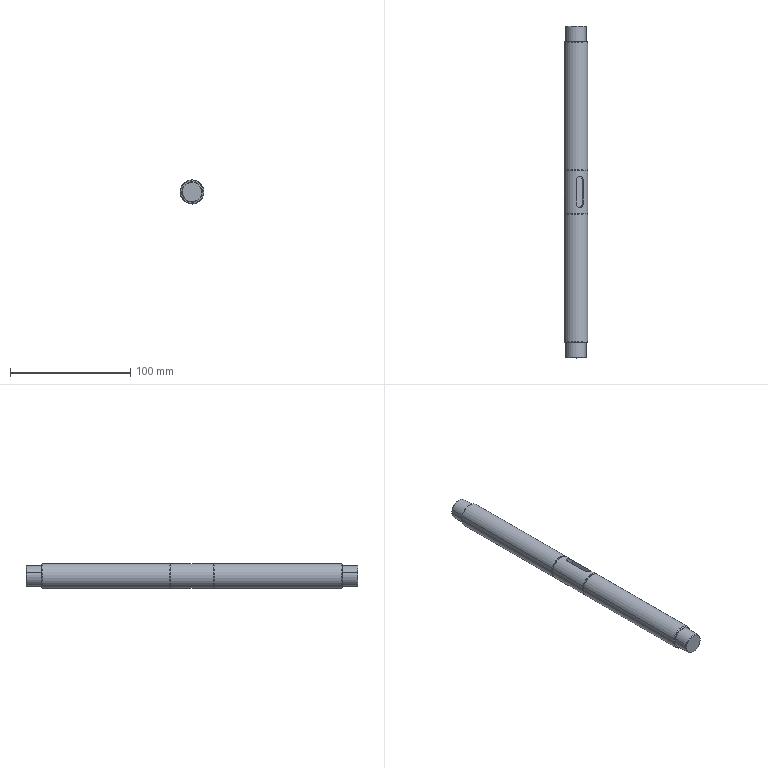Component | SolidWorks | CTM-T-12-D-GD-03-1 | 1 solid | 36 faces | box 20 x 276 x 20 mm | volume 83848 mm3 | cylinder 17 | plane 11 | cone 8 | commonest cylinder face diameters 20 x6 17 x4 19 x4 6 x3 | material 45
build123d program:
from build123d import *

# Parameters (mm, degrees)
SKETCH1_R           = 10
BOSS_EXTRUDE1_DEPTH = 125
SKETCH2_R           = 8.5
BOSS_EXTRUDE2_DEPTH = 13
BOSS_EXTRUDE3_START = 13
SKETCH3_R           = 8.5
BOSS_EXTRUDE3_DEPTH = 13
CUT_EXTRUDE2_DEPTH  = 3.5
CHAMFER1_SIZE       = 0.5
CHAMFER2_SIZE       = 0.5
SKETCH8_R           = 10
SKETCH8_R_2         = 9.5
CUT_EXTRUDE3_DEPTH  = 1.1


with BuildPart() as part:
    # Sketch1 → Boss-Extrude1 (new, symmetric)
    with BuildSketch(Plane.XY):
        Circle(SKETCH1_R)
    extrude(amount=BOSS_EXTRUDE1_DEPTH, both=True)

    # Sketch2 → Boss-Extrude2 (add)
    with BuildSketch(Plane(origin=(0, 0, -125), x_dir=(-1, 0, 0), z_dir=(0, 0, -1))):
        with Locations(Location((0, 0, 0), (0, 0, 180))):
            Circle(SKETCH2_R)
    extrude(amount=BOSS_EXTRUDE2_DEPTH)

    # Sketch3 → Boss-Extrude3 (add)
    with BuildSketch(Plane.XY.offset(125).offset(BOSS_EXTRUDE3_START)):
        Circle(SKETCH3_R)
    extrude(amount=-BOSS_EXTRUDE3_DEPTH)

    # Sketch7 → Cut-Extrude2 (cut)
    with BuildSketch(Plane(origin=(0, 10, 0), x_dir=(-1, 0, 0), z_dir=(0, 1, 0))):
        with BuildLine():
            Line((3, 10), (3, -10))
            ThreePointArc((3, -10), (0, -13), (-3, -10))
            Line((-3, -10), (-3, 10))
            ThreePointArc((-3, 10), (0, 13), (3, 10))
        make_face()
    extrude(amount=-CUT_EXTRUDE2_DEPTH, mode=Mode.SUBTRACT)

    # Chamfer1
    chamfer1_edges = [part.edges().sort_by_distance(p)[0] for p in [
        (-8.5, 0, 138),
        (-8.5, 0, -138),
    ]]
    chamfer(chamfer1_edges, length=CHAMFER1_SIZE)

    # Chamfer2
    chamfer2_edges = [part.edges().sort_by_distance(p)[0] for p in [
        (-10, 0, -125),
        (-10, 0, 125),
    ]]
    chamfer(chamfer2_edges, length=CHAMFER2_SIZE)

    # Sketch8 → Cut-Extrude3 (cut)
    with BuildSketch(Plane.XY.offset(18.65)):
        Circle(SKETCH8_R)
        Circle(SKETCH8_R_2, mode=Mode.SUBTRACT)
    cut_extrude3 = extrude(amount=-CUT_EXTRUDE3_DEPTH, mode=Mode.SUBTRACT)

    # Mirror1: Cut-Extrude3 across plane
    add(cut_extrude3.mirror(Plane.XY), mode=Mode.SUBTRACT)


solid = part.part

# Placed as in the assembly
solid = solid.moved(Location((40.4, -145, 35), (-90, 0, -160.666)))
STEP:
#1=CARTESIAN_POINT('',(1.962,-4.974,1.248));
#2=VERTEX_POINT('',#1);
#3=CARTESIAN_POINT('',(1.219,-4.974,1.508));
#4=VERTEX_POINT('',#3);
#5=CARTESIAN_POINT('',(1.591,-4.974,1.378));
#6=DIRECTION('',(-0.,-1.,-0.));
#7=DIRECTION('',(0.9436,0.,-0.3311));
#8=AXIS2_PLACEMENT_3D('',#5,#6,#7);
#9=CIRCLE('',#8,0.3937);
#10=EDGE_CURVE('',#2,#4,#9,.T.);
#11=ORIENTED_EDGE('',*,*,#10,.F.);
#12=CARTESIAN_POINT('',(1.962,-0.8071,1.248));
#13=VERTEX_POINT('',#12);
#14=CARTESIAN_POINT('',(1.962,-10.63,1.248));
#15=DIRECTION('',(0.,1.,0.));
#16=VECTOR('',#15,39.37);
#17=LINE('',#14,#16);
#18=EDGE_CURVE('',#2,#13,#17,.T.);
#19=ORIENTED_EDGE('',*,*,#18,.T.);
#20=CARTESIAN_POINT('',(1.219,-0.8071,1.508));
#21=VERTEX_POINT('',#20);
#22=CARTESIAN_POINT('',(1.591,-0.8071,1.378));
#23=DIRECTION('',(-0.,-1.,-0.));
#24=DIRECTION('',(0.9436,0.,-0.3311));
#25=AXIS2_PLACEMENT_3D('',#22,#23,#24);
#26=CIRCLE('',#25,0.3937);
#27=EDGE_CURVE('',#13,#21,#26,.T.);
#28=ORIENTED_EDGE('',*,*,#27,.T.);
#29=CARTESIAN_POINT('',(1.219,-10.63,1.508));
#30=DIRECTION('',(0.,1.,0.));
#31=VECTOR('',#30,39.37);
#32=LINE('',#29,#31);
#33=EDGE_CURVE('',#4,#21,#32,.T.);
#34=ORIENTED_EDGE('',*,*,#33,.F.);
#35=EDGE_LOOP('',(#11,#19,#28,#34));
#36=FACE_OUTER_BOUND('',#35,.T.);
#37=CARTESIAN_POINT('',(1.591,-10.63,1.378));
#38=DIRECTION('',(0.,1.,0.));
#39=DIRECTION('',(-0.9436,0.,0.3311));
#40=AXIS2_PLACEMENT_3D('',#37,#38,#39);
#41=CYLINDRICAL_SURFACE('',#40,0.3937);
#42=ADVANCED_FACE('',(#36),#41,.T.);
#43=CARTESIAN_POINT('',(1.238,-0.7874,1.502));
#44=VERTEX_POINT('',#43);
#45=CARTESIAN_POINT('',(1.943,-0.7874,1.254));
#46=VERTEX_POINT('',#45);
#47=CARTESIAN_POINT('',(1.591,-0.7874,1.378));
#48=DIRECTION('',(0.,1.,0.));
#49=DIRECTION('',(0.9436,0.,-0.3311));
#50=AXIS2_PLACEMENT_3D('',#47,#48,#49);
#51=CIRCLE('',#50,0.374);
#52=EDGE_CURVE('',#44,#46,#51,.T.);
#53=ORIENTED_EDGE('',*,*,#52,.F.);
#54=CARTESIAN_POINT('',(1.219,-0.8071,1.508));
#55=DIRECTION('',(-0.6672,-0.7071,0.2341));
#56=VECTOR('',#55,39.37);
#57=LINE('',#54,#56);
#58=EDGE_CURVE('',#44,#21,#57,.T.);
#59=ORIENTED_EDGE('',*,*,#58,.T.);
#60=ORIENTED_EDGE('',*,*,#27,.F.);
#61=CARTESIAN_POINT('',(1.962,-0.8071,1.248));
#62=DIRECTION('',(0.6672,-0.7071,-0.2341));
#63=VECTOR('',#62,39.37);
#64=LINE('',#61,#63);
#65=EDGE_CURVE('',#46,#13,#64,.T.);
#66=ORIENTED_EDGE('',*,*,#65,.F.);
#67=EDGE_LOOP('',(#53,#59,#60,#66));
#68=FACE_OUTER_BOUND('',#67,.T.);
#69=CARTESIAN_POINT('',(1.591,-0.8071,1.378));
#70=DIRECTION('',(-0.,-1.,-0.));
#71=DIRECTION('',(0.9436,0.,-0.3311));
#72=AXIS2_PLACEMENT_3D('',#69,#70,#71);
#73=CONICAL_SURFACE('',#72,0.3937,0.7854);
#74=ADVANCED_FACE('',(#68),#73,.T.);
#75=CARTESIAN_POINT('',(1.906,-0.2953,1.267));
#76=VERTEX_POINT('',#75);
#77=CARTESIAN_POINT('',(1.275,-0.2953,1.489));
#78=VERTEX_POINT('',#77);
#79=CARTESIAN_POINT('',(1.591,-0.2953,1.378));
#80=DIRECTION('',(-0.,-1.,-0.));
#81=DIRECTION('',(-0.9436,0.,0.3311));
#82=AXIS2_PLACEMENT_3D('',#79,#80,#81);
#83=CIRCLE('',#82,0.3346);
#84=EDGE_CURVE('',#76,#78,#83,.T.);
#85=ORIENTED_EDGE('',*,*,#84,.T.);
#86=CARTESIAN_POINT('',(1.275,-0.7874,1.489));
#87=VERTEX_POINT('',#86);
#88=CARTESIAN_POINT('',(1.275,-0.2756,1.489));
#89=DIRECTION('',(-0.,-1.,-0.));
#90=VECTOR('',#89,39.37);
#91=LINE('',#88,#90);
#92=EDGE_CURVE('',#78,#87,#91,.T.);
#93=ORIENTED_EDGE('',*,*,#92,.T.);
#94=CARTESIAN_POINT('',(1.906,-0.7874,1.267));
#95=VERTEX_POINT('',#94);
#96=CARTESIAN_POINT('',(1.591,-0.7874,1.378));
#97=DIRECTION('',(0.,1.,0.));
#98=DIRECTION('',(0.9436,0.,-0.3311));
#99=AXIS2_PLACEMENT_3D('',#96,#97,#98);
#100=CIRCLE('',#99,0.3346);
#101=EDGE_CURVE('',#87,#95,#100,.T.);
#102=ORIENTED_EDGE('',*,*,#101,.T.);
#103=CARTESIAN_POINT('',(1.906,-0.2756,1.267));
#104=DIRECTION('',(-0.,-1.,-0.));
#105=VECTOR('',#104,39.37);
#106=LINE('',#103,#105);
#107=EDGE_CURVE('',#76,#95,#106,.T.);
#108=ORIENTED_EDGE('',*,*,#107,.F.);
#109=EDGE_LOOP('',(#85,#93,#102,#108));
#110=FACE_OUTER_BOUND('',#109,.T.);
#111=CARTESIAN_POINT('',(1.591,-0.2756,1.378));
#112=DIRECTION('',(-0.,-1.,-0.));
#113=DIRECTION('',(0.9436,-0.,-0.3311));
#114=AXIS2_PLACEMENT_3D('',#111,#112,#113);
#115=CYLINDRICAL_SURFACE('',#114,0.3346);
#116=ADVANCED_FACE('',(#110),#115,.T.);
#117=CARTESIAN_POINT('',(1.293,-0.2756,1.482));
#118=VERTEX_POINT('',#117);
#119=CARTESIAN_POINT('',(1.888,-0.2756,1.274));
#120=VERTEX_POINT('',#119);
#121=CARTESIAN_POINT('',(1.591,-0.2756,1.378));
#122=DIRECTION('',(0.,1.,0.));
#123=DIRECTION('',(-0.9436,0.,0.3311));
#124=AXIS2_PLACEMENT_3D('',#121,#122,#123);
#125=CIRCLE('',#124,0.315);
#126=EDGE_CURVE('',#118,#120,#125,.T.);
#127=ORIENTED_EDGE('',*,*,#126,.F.);
#128=CARTESIAN_POINT('',(1.293,-0.2756,1.482));
#129=DIRECTION('',(-0.6672,-0.7071,0.2341));
#130=VECTOR('',#129,39.37);
#131=LINE('',#128,#130);
#132=EDGE_CURVE('',#118,#78,#131,.T.);
#133=ORIENTED_EDGE('',*,*,#132,.T.);
#134=ORIENTED_EDGE('',*,*,#84,.F.);
#135=CARTESIAN_POINT('',(1.888,-0.2756,1.274));
#136=DIRECTION('',(0.6672,-0.7071,-0.2341));
#137=VECTOR('',#136,39.37);
#138=LINE('',#135,#137);
#139=EDGE_CURVE('',#120,#76,#138,.T.);
#140=ORIENTED_EDGE('',*,*,#139,.F.);
#141=EDGE_LOOP('',(#127,#133,#134,#140));
#142=FACE_OUTER_BOUND('',#141,.T.);
#143=CARTESIAN_POINT('',(1.591,-0.2756,1.378));
#144=DIRECTION('',(-0.,-1.,-0.));
#145=DIRECTION('',(0.9436,-0.,-0.3311));
#146=AXIS2_PLACEMENT_3D('',#143,#144,#145);
#147=CONICAL_SURFACE('',#146,0.315,0.7854);
#148=ADVANCED_FACE('',(#142),#147,.T.);
#149=CARTESIAN_POINT('',(1.943,-5.018,1.254));
#150=VERTEX_POINT('',#149);
#151=CARTESIAN_POINT('',(1.238,-5.018,1.502));
#152=VERTEX_POINT('',#151);
#153=CARTESIAN_POINT('',(1.591,-5.018,1.378));
#154=DIRECTION('',(-0.,-1.,-0.));
#155=DIRECTION('',(0.9436,0.,-0.3311));
#156=AXIS2_PLACEMENT_3D('',#153,#154,#155);
#157=CIRCLE('',#156,0.374);
#158=EDGE_CURVE('',#150,#152,#157,.T.);
#159=ORIENTED_EDGE('',*,*,#158,.F.);
#160=CARTESIAN_POINT('',(1.943,-4.974,1.254));
#161=VERTEX_POINT('',#160);
#162=CARTESIAN_POINT('',(1.943,-5.018,1.254));
#163=DIRECTION('',(0.,1.,0.));
#164=VECTOR('',#163,39.37);
#165=LINE('',#162,#164);
#166=EDGE_CURVE('',#150,#161,#165,.T.);
#167=ORIENTED_EDGE('',*,*,#166,.T.);
#168=CARTESIAN_POINT('',(1.238,-4.974,1.502));
#169=VERTEX_POINT('',#168);
#170=CARTESIAN_POINT('',(1.591,-4.974,1.378));
#171=DIRECTION('',(-0.,-1.,-0.));
#172=DIRECTION('',(0.9436,0.,-0.3311));
#173=AXIS2_PLACEMENT_3D('',#170,#171,#172);
#174=CIRCLE('',#173,0.374);
#175=EDGE_CURVE('',#161,#169,#174,.T.);
#176=ORIENTED_EDGE('',*,*,#175,.T.);
#177=CARTESIAN_POINT('',(1.238,-5.018,1.502));
#178=DIRECTION('',(0.,1.,0.));
#179=VECTOR('',#178,39.37);
#180=LINE('',#177,#179);
#181=EDGE_CURVE('',#152,#169,#180,.T.);
#182=ORIENTED_EDGE('',*,*,#181,.F.);
#183=EDGE_LOOP('',(#159,#167,#176,#182));
#184=FACE_OUTER_BOUND('',#183,.T.);
#185=CARTESIAN_POINT('',(1.591,-5.018,1.378));
#186=DIRECTION('',(0.,1.,0.));
#187=DIRECTION('',(-0.9436,0.,0.3311));
#188=AXIS2_PLACEMENT_3D('',#185,#186,#187);
#189=CYLINDRICAL_SURFACE('',#188,0.374);
#190=ADVANCED_FACE('',(#184),#189,.T.);
#191=CARTESIAN_POINT('',(1.219,-10.61,1.508));
#192=VERTEX_POINT('',#191);
#193=CARTESIAN_POINT('',(1.962,-10.61,1.248));
#194=VERTEX_POINT('',#193);
#195=CARTESIAN_POINT('',(1.591,-10.61,1.378));
#196=DIRECTION('',(0.,1.,0.));
#197=DIRECTION('',(0.9436,0.,-0.3311));
#198=AXIS2_PLACEMENT_3D('',#195,#196,#197);
#199=CIRCLE('',#198,0.3937);
#200=EDGE_CURVE('',#192,#194,#199,.T.);
#201=ORIENTED_EDGE('',*,*,#200,.T.);
#202=CARTESIAN_POINT('',(1.962,-6.443,1.248));
#203=VERTEX_POINT('',#202);
#204=CARTESIAN_POINT('',(1.962,-10.63,1.248));
#205=DIRECTION('',(0.,1.,0.));
#206=VECTOR('',#205,39.37);
#207=LINE('',#204,#206);
#208=EDGE_CURVE('',#194,#203,#207,.T.);
#209=ORIENTED_EDGE('',*,*,#208,.T.);
#210=CARTESIAN_POINT('',(1.219,-6.443,1.508));
#211=VERTEX_POINT('',#210);
#212=CARTESIAN_POINT('',(1.591,-6.443,1.378));
#213=DIRECTION('',(-0.,-1.,-0.));
#214=DIRECTION('',(0.9436,0.,-0.3311));
#215=AXIS2_PLACEMENT_3D('',#212,#213,#214);
#216=CIRCLE('',#215,0.3937);
#217=EDGE_CURVE('',#203,#211,#216,.T.);
#218=ORIENTED_EDGE('',*,*,#217,.T.);
#219=CARTESIAN_POINT('',(1.219,-10.63,1.508));
#220=DIRECTION('',(0.,1.,0.));
#221=VECTOR('',#220,39.37);
#222=LINE('',#219,#221);
#223=EDGE_CURVE('',#192,#211,#222,.T.);
#224=ORIENTED_EDGE('',*,*,#223,.F.);
#225=EDGE_LOOP('',(#201,#209,#218,#224));
#226=FACE_OUTER_BOUND('',#225,.T.);
#227=CARTESIAN_POINT('',(1.591,-10.63,1.378));
#228=DIRECTION('',(0.,1.,0.));
#229=DIRECTION('',(-0.9436,0.,0.3311));
#230=AXIS2_PLACEMENT_3D('',#227,#228,#229);
#231=CYLINDRICAL_SURFACE('',#230,0.3937);
#232=ADVANCED_FACE('',(#226),#231,.T.);
#233=CARTESIAN_POINT('',(1.943,-10.63,1.254));
#234=VERTEX_POINT('',#233);
#235=CARTESIAN_POINT('',(1.238,-10.63,1.502));
#236=VERTEX_POINT('',#235);
#237=CARTESIAN_POINT('',(1.591,-10.63,1.378));
#238=DIRECTION('',(-0.,-1.,-0.));
#239=DIRECTION('',(0.9436,0.,-0.3311));
#240=AXIS2_PLACEMENT_3D('',#237,#238,#239);
#241=CIRCLE('',#240,0.374);
#242=EDGE_CURVE('',#234,#236,#241,.T.);
#243=ORIENTED_EDGE('',*,*,#242,.F.);
#244=CARTESIAN_POINT('',(1.943,-10.63,1.254));
#245=DIRECTION('',(0.6672,0.7071,-0.2341));
#246=VECTOR('',#245,39.37);
#247=LINE('',#244,#246);
#248=EDGE_CURVE('',#234,#194,#247,.T.);
#249=ORIENTED_EDGE('',*,*,#248,.T.);
#250=ORIENTED_EDGE('',*,*,#200,.F.);
#251=CARTESIAN_POINT('',(1.238,-10.63,1.502));
#252=DIRECTION('',(-0.6672,0.7071,0.2341));
#253=VECTOR('',#252,39.37);
#254=LINE('',#251,#253);
#255=EDGE_CURVE('',#236,#192,#254,.T.);
#256=ORIENTED_EDGE('',*,*,#255,.F.);
#257=EDGE_LOOP('',(#243,#249,#250,#256));
#258=FACE_OUTER_BOUND('',#257,.T.);
#259=CARTESIAN_POINT('',(1.591,-10.63,1.378));
#260=DIRECTION('',(0.,1.,0.));
#261=DIRECTION('',(-0.9436,0.,0.3311));
#262=AXIS2_PLACEMENT_3D('',#259,#260,#261);
#263=CONICAL_SURFACE('',#262,0.374,0.7854);
#264=ADVANCED_FACE('',(#258),#263,.T.);
#265=CARTESIAN_POINT('',(1.275,-11.122,1.489));
#266=VERTEX_POINT('',#265);
#267=CARTESIAN_POINT('',(1.906,-11.122,1.267));
#268=VERTEX_POINT('',#267);
#269=CARTESIAN_POINT('',(1.591,-11.122,1.378));
#270=DIRECTION('',(0.,1.,0.));
#271=DIRECTION('',(0.9436,0.,-0.3311));
#272=AXIS2_PLACEMENT_3D('',#269,#270,#271);
#273=CIRCLE('',#272,0.3346);
#274=EDGE_CURVE('',#266,#268,#273,.T.);
#275=ORIENTED_EDGE('',*,*,#274,.T.);
#276=CARTESIAN_POINT('',(1.906,-10.63,1.267));
#277=VERTEX_POINT('',#276);
#278=CARTESIAN_POINT('',(1.906,-11.142,1.267));
#279=DIRECTION('',(0.,1.,0.));
#280=VECTOR('',#279,39.37);
#281=LINE('',#278,#280);
#282=EDGE_CURVE('',#268,#277,#281,.T.);
#283=ORIENTED_EDGE('',*,*,#282,.T.);
#284=CARTESIAN_POINT('',(1.275,-10.63,1.489));
#285=VERTEX_POINT('',#284);
#286=CARTESIAN_POINT('',(1.591,-10.63,1.378));
#287=DIRECTION('',(-0.,-1.,-0.));
#288=DIRECTION('',(0.9436,0.,-0.3311));
#289=AXIS2_PLACEMENT_3D('',#286,#287,#288);
#290=CIRCLE('',#289,0.3346);
#291=EDGE_CURVE('',#277,#285,#290,.T.);
#292=ORIENTED_EDGE('',*,*,#291,.T.);
#293=CARTESIAN_POINT('',(1.275,-11.142,1.489));
#294=DIRECTION('',(0.,1.,0.));
#295=VECTOR('',#294,39.37);
#296=LINE('',#293,#295);
#297=EDGE_CURVE('',#266,#285,#296,.T.);
#298=ORIENTED_EDGE('',*,*,#297,.F.);
#299=EDGE_LOOP('',(#275,#283,#292,#298));
#300=FACE_OUTER_BOUND('',#299,.T.);
#301=CARTESIAN_POINT('',(1.591,-11.142,1.378));
#302=DIRECTION('',(0.,1.,0.));
#303=DIRECTION('',(-0.9436,0.,0.3311));
#304=AXIS2_PLACEMENT_3D('',#301,#302,#303);
#305=CYLINDRICAL_SURFACE('',#304,0.3346);
#306=ADVANCED_FACE('',(#300),#305,.T.);
#307=CARTESIAN_POINT('',(1.888,-11.142,1.274));
#308=VERTEX_POINT('',#307);
#309=CARTESIAN_POINT('',(1.293,-11.142,1.482));
#310=VERTEX_POINT('',#309);
#311=CARTESIAN_POINT('',(1.591,-11.142,1.378));
#312=DIRECTION('',(-0.,-1.,-0.));
#313=DIRECTION('',(0.9436,0.,-0.3311));
#314=AXIS2_PLACEMENT_3D('',#311,#312,#313);
#315=CIRCLE('',#314,0.315);
#316=EDGE_CURVE('',#308,#310,#315,.T.);
#317=ORIENTED_EDGE('',*,*,#316,.F.);
#318=CARTESIAN_POINT('',(1.888,-11.142,1.274));
#319=DIRECTION('',(0.6672,0.7071,-0.2341));
#320=VECTOR('',#319,39.37);
#321=LINE('',#318,#320);
#322=EDGE_CURVE('',#308,#268,#321,.T.);
#323=ORIENTED_EDGE('',*,*,#322,.T.);
#324=ORIENTED_EDGE('',*,*,#274,.F.);
#325=CARTESIAN_POINT('',(1.293,-11.142,1.482));
#326=DIRECTION('',(-0.6672,0.7071,0.2341));
#327=VECTOR('',#326,39.37);
#328=LINE('',#325,#327);
#329=EDGE_CURVE('',#310,#266,#328,.T.);
#330=ORIENTED_EDGE('',*,*,#329,.F.);
#331=EDGE_LOOP('',(#317,#323,#324,#330));
#332=FACE_OUTER_BOUND('',#331,.T.);
#333=CARTESIAN_POINT('',(1.591,-11.142,1.378));
#334=DIRECTION('',(0.,1.,0.));
#335=DIRECTION('',(-0.9436,0.,0.3311));
#336=AXIS2_PLACEMENT_3D('',#333,#334,#335);
#337=CONICAL_SURFACE('',#336,0.315,0.7854);
#338=ADVANCED_FACE('',(#332),#337,.T.);
#339=CARTESIAN_POINT('',(1.943,-6.4,1.254));
#340=VERTEX_POINT('',#339);
#341=CARTESIAN_POINT('',(1.238,-6.4,1.502));
#342=VERTEX_POINT('',#341);
#343=CARTESIAN_POINT('',(1.591,-6.4,1.378));
#344=DIRECTION('',(-0.,-1.,-0.));
#345=DIRECTION('',(0.9436,0.,-0.3311));
#346=AXIS2_PLACEMENT_3D('',#343,#344,#345);
#347=CIRCLE('',#346,0.374);
#348=EDGE_CURVE('',#340,#342,#347,.T.);
#349=ORIENTED_EDGE('',*,*,#348,.T.);
#350=CARTESIAN_POINT('',(1.238,-6.443,1.502));
#351=VERTEX_POINT('',#350);
#352=CARTESIAN_POINT('',(1.238,-6.4,1.502));
#353=DIRECTION('',(-0.,-1.,-0.));
#354=VECTOR('',#353,39.37);
#355=LINE('',#352,#354);
#356=EDGE_CURVE('',#342,#351,#355,.T.);
#357=ORIENTED_EDGE('',*,*,#356,.T.);
#358=CARTESIAN_POINT('',(1.943,-6.443,1.254));
#359=VERTEX_POINT('',#358);
#360=CARTESIAN_POINT('',(1.591,-6.443,1.378));
#361=DIRECTION('',(-0.,-1.,-0.));
#362=DIRECTION('',(0.9436,0.,-0.3311));
#363=AXIS2_PLACEMENT_3D('',#360,#361,#362);
#364=CIRCLE('',#363,0.374);
#365=EDGE_CURVE('',#359,#351,#364,.T.);
#366=ORIENTED_EDGE('',*,*,#365,.F.);
#367=CARTESIAN_POINT('',(1.943,-6.4,1.254));
#368=DIRECTION('',(-0.,-1.,-0.));
#369=VECTOR('',#368,39.37);
#370=LINE('',#367,#369);
#371=EDGE_CURVE('',#340,#359,#370,.T.);
#372=ORIENTED_EDGE('',*,*,#371,.F.);
#373=EDGE_LOOP('',(#349,#357,#366,#372));
#374=FACE_OUTER_BOUND('',#373,.T.);
#375=CARTESIAN_POINT('',(1.591,-6.4,1.378));
#376=DIRECTION('',(-0.,-1.,-0.));
#377=DIRECTION('',(0.9436,0.,-0.3311));
#378=AXIS2_PLACEMENT_3D('',#375,#376,#377);
#379=CYLINDRICAL_SURFACE('',#378,0.374);
#380=ADVANCED_FACE('',(#374),#379,.T.);
#381=CARTESIAN_POINT('',(1.675,-6.22,1.619));
#382=VERTEX_POINT('',#381);
#383=CARTESIAN_POINT('',(1.787,-6.102,1.58));
#384=VERTEX_POINT('',#383);
#385=CARTESIAN_POINT('',(1.675,-6.102,1.619));
#386=DIRECTION('',(0.3311,-0.,0.9436));
#387=DIRECTION('',(0.,-1.,0.));
#388=AXIS2_PLACEMENT_3D('',#385,#386,#387);
#389=CIRCLE('',#388,0.1181);
#390=EDGE_CURVE('',#382,#384,#389,.T.);
#391=ORIENTED_EDGE('',*,*,#390,.F.);
#392=CARTESIAN_POINT('',(1.721,-6.22,1.749));
#393=VERTEX_POINT('',#392);
#394=CARTESIAN_POINT('',(1.675,-6.22,1.619));
#395=DIRECTION('',(0.3311,-0.,0.9436));
#396=VECTOR('',#395,39.37);
#397=LINE('',#394,#396);
#398=EDGE_CURVE('',#382,#393,#397,.T.);
#399=ORIENTED_EDGE('',*,*,#398,.T.);
#400=CARTESIAN_POINT('',(1.826,-6.102,1.693));
#401=VERTEX_POINT('',#400);
#402=CARTESIAN_POINT('',(1.826,-6.102,1.693));
#403=CARTESIAN_POINT('',(1.826,-6.11,1.693));
#404=CARTESIAN_POINT('',(1.826,-6.118,1.694));
#405=CARTESIAN_POINT('',(1.823,-6.133,1.696));
#406=CARTESIAN_POINT('',(1.821,-6.141,1.697));
#407=CARTESIAN_POINT('',(1.816,-6.155,1.701));
#408=CARTESIAN_POINT('',(1.813,-6.162,1.703));
#409=CARTESIAN_POINT('',(1.806,-6.174,1.708));
#410=CARTESIAN_POINT('',(1.801,-6.181,1.71));
#411=CARTESIAN_POINT('',(1.787,-6.197,1.719));
#412=CARTESIAN_POINT('',(1.776,-6.206,1.726));
#413=CARTESIAN_POINT('',(1.756,-6.214,1.735));
#414=CARTESIAN_POINT('',(1.75,-6.217,1.738));
#415=CARTESIAN_POINT('',(1.735,-6.22,1.744));
#416=CARTESIAN_POINT('',(1.728,-6.22,1.747));
#417=CARTESIAN_POINT('',(1.721,-6.22,1.749));
#418=B_SPLINE_CURVE_WITH_KNOTS('',3,(#402,#403,#404,#405,#406,#407,#408,#409,#410,#411,#412,#413,#414,#415,#416,#417),.UNSPECIFIED.,.F.,.F.,(4,2,2,2,2,2,2,4),(0.,0.0005898,0.00118,0.001769,0.002359,0.003539,0.004128,0.004718),.UNSPECIFIED.);
#419=EDGE_CURVE('',#401,#393,#418,.T.);
#420=ORIENTED_EDGE('',*,*,#419,.F.);
#421=CARTESIAN_POINT('',(1.787,-6.102,1.58));
#422=DIRECTION('',(0.3311,-0.,0.9436));
#423=VECTOR('',#422,39.37);
#424=LINE('',#421,#423);
#425=EDGE_CURVE('',#384,#401,#424,.T.);
#426=ORIENTED_EDGE('',*,*,#425,.F.);
#427=EDGE_LOOP('',(#391,#399,#420,#426));
#428=FACE_OUTER_BOUND('',#427,.T.);
#429=CARTESIAN_POINT('',(1.675,-6.102,1.619));
#430=DIRECTION('',(0.3311,-0.,0.9436));
#431=DIRECTION('',(0.,-1.,0.));
#432=AXIS2_PLACEMENT_3D('',#429,#430,#431);
#433=CYLINDRICAL_SURFACE('',#432,0.1181);
#434=ADVANCED_FACE('',(#428),#433,.F.);
#435=CARTESIAN_POINT('',(1.603,-6.102,1.771));
#436=VERTEX_POINT('',#435);
#437=CARTESIAN_POINT('',(1.603,-5.315,1.771));
#438=VERTEX_POINT('',#437);
#439=CARTESIAN_POINT('',(1.603,-10.63,1.771));
#440=DIRECTION('',(0.,1.,0.));
#441=VECTOR('',#440,39.37);
#442=LINE('',#439,#441);
#443=EDGE_CURVE('',#436,#438,#442,.T.);
#444=ORIENTED_EDGE('',*,*,#443,.T.);
#445=CARTESIAN_POINT('',(1.826,-5.315,1.693));
#446=VERTEX_POINT('',#445);
#447=CARTESIAN_POINT('',(1.603,-5.315,1.771));
#448=CARTESIAN_POINT('',(1.603,-5.307,1.771));
#449=CARTESIAN_POINT('',(1.604,-5.299,1.771));
#450=CARTESIAN_POINT('',(1.607,-5.284,1.771));
#451=CARTESIAN_POINT('',(1.61,-5.277,1.771));
#452=CARTESIAN_POINT('',(1.616,-5.262,1.771));
#453=CARTESIAN_POINT('',(1.62,-5.256,1.771));
#454=CARTESIAN_POINT('',(1.629,-5.243,1.77));
#455=CARTESIAN_POINT('',(1.634,-5.237,1.769));
#456=CARTESIAN_POINT('',(1.65,-5.221,1.767));
#457=CARTESIAN_POINT('',(1.663,-5.212,1.765));
#458=CARTESIAN_POINT('',(1.684,-5.203,1.76));
#459=CARTESIAN_POINT('',(1.691,-5.201,1.759));
#460=CARTESIAN_POINT('',(1.706,-5.198,1.754));
#461=CARTESIAN_POINT('',(1.713,-5.197,1.752));
#462=CARTESIAN_POINT('',(1.728,-5.197,1.747));
#463=CARTESIAN_POINT('',(1.735,-5.198,1.744));
#464=CARTESIAN_POINT('',(1.749,-5.201,1.738));
#465=CARTESIAN_POINT('',(1.756,-5.203,1.735));
#466=CARTESIAN_POINT('',(1.769,-5.209,1.729));
#467=CARTESIAN_POINT('',(1.775,-5.213,1.726));
#468=CARTESIAN_POINT('',(1.787,-5.221,1.719));
#469=CARTESIAN_POINT('',(1.792,-5.226,1.716));
#470=CARTESIAN_POINT('',(1.801,-5.237,1.71));
#471=CARTESIAN_POINT('',(1.806,-5.243,1.708));
#472=CARTESIAN_POINT('',(1.813,-5.256,1.703));
#473=CARTESIAN_POINT('',(1.816,-5.262,1.701));
#474=CARTESIAN_POINT('',(1.821,-5.277,1.697));
#475=CARTESIAN_POINT('',(1.823,-5.284,1.696));
#476=CARTESIAN_POINT('',(1.826,-5.299,1.694));
#477=CARTESIAN_POINT('',(1.826,-5.307,1.693));
#478=CARTESIAN_POINT('',(1.826,-5.315,1.693));
#479=B_SPLINE_CURVE_WITH_KNOTS('',3,(#447,#448,#449,#450,#451,#452,#453,#454,#455,#456,#457,#458,#459,#460,#461,#462,#463,#464,#465,#466,#467,#468,#469,#470,#471,#472,#473,#474,#475,#476,#477,#478),.UNSPECIFIED.,.F.,.F.,(4,2,2,2,2,2,2,2,2,2,2,2,2,2,2,4),(0.,0.0005894,0.001179,0.001768,0.002358,0.003536,0.004126,0.004715,0.005305,0.005894,0.006484,0.007073,0.007662,0.008252,0.008841,0.009431),.UNSPECIFIED.);
#480=EDGE_CURVE('',#438,#446,#479,.T.);
#481=ORIENTED_EDGE('',*,*,#480,.T.);
#482=CARTESIAN_POINT('',(1.826,-10.63,1.693));
#483=DIRECTION('',(-0.,-1.,-0.));
#484=VECTOR('',#483,39.37);
#485=LINE('',#482,#484);
#486=EDGE_CURVE('',#446,#401,#485,.T.);
#487=ORIENTED_EDGE('',*,*,#486,.T.);
#488=ORIENTED_EDGE('',*,*,#419,.T.);
#489=CARTESIAN_POINT('',(1.721,-6.22,1.749));
#490=CARTESIAN_POINT('',(1.714,-6.22,1.752));
#491=CARTESIAN_POINT('',(1.706,-6.22,1.754));
#492=CARTESIAN_POINT('',(1.691,-6.217,1.759));
#493=CARTESIAN_POINT('',(1.684,-6.214,1.76));
#494=CARTESIAN_POINT('',(1.67,-6.208,1.764));
#495=CARTESIAN_POINT('',(1.663,-6.205,1.765));
#496=CARTESIAN_POINT('',(1.651,-6.196,1.767));
#497=CARTESIAN_POINT('',(1.645,-6.191,1.768));
#498=CARTESIAN_POINT('',(1.634,-6.18,1.769));
#499=CARTESIAN_POINT('',(1.629,-6.175,1.77));
#500=CARTESIAN_POINT('',(1.62,-6.162,1.771));
#501=CARTESIAN_POINT('',(1.616,-6.155,1.771));
#502=CARTESIAN_POINT('',(1.61,-6.141,1.771));
#503=CARTESIAN_POINT('',(1.607,-6.133,1.771));
#504=CARTESIAN_POINT('',(1.604,-6.118,1.771));
#505=CARTESIAN_POINT('',(1.603,-6.11,1.771));
#506=CARTESIAN_POINT('',(1.603,-6.102,1.771));
#507=B_SPLINE_CURVE_WITH_KNOTS('',3,(#489,#490,#491,#492,#493,#494,#495,#496,#497,#498,#499,#500,#501,#502,#503,#504,#505,#506),.UNSPECIFIED.,.F.,.F.,(4,2,2,2,2,2,2,2,4),(0.004718,0.005307,0.005896,0.006485,0.007074,0.007663,0.008252,0.008842,0.009431),.UNSPECIFIED.);
#508=EDGE_CURVE('',#393,#436,#507,.T.);
#509=ORIENTED_EDGE('',*,*,#508,.T.);
#510=EDGE_LOOP('',(#444,#481,#487,#488,#509));
#511=FACE_BOUND('',#510,.T.);
#512=CARTESIAN_POINT('',(1.962,-6.4,1.248));
#513=VERTEX_POINT('',#512);
#514=CARTESIAN_POINT('',(1.219,-6.4,1.508));
#515=VERTEX_POINT('',#514);
#516=CARTESIAN_POINT('',(1.591,-6.4,1.378));
#517=DIRECTION('',(-0.,-1.,-0.));
#518=DIRECTION('',(0.9436,0.,-0.3311));
#519=AXIS2_PLACEMENT_3D('',#516,#517,#518);
#520=CIRCLE('',#519,0.3937);
#521=EDGE_CURVE('',#513,#515,#520,.T.);
#522=ORIENTED_EDGE('',*,*,#521,.F.);
#523=CARTESIAN_POINT('',(1.962,-5.018,1.248));
#524=VERTEX_POINT('',#523);
#525=CARTESIAN_POINT('',(1.962,-10.63,1.248));
#526=DIRECTION('',(0.,1.,0.));
#527=VECTOR('',#526,39.37);
#528=LINE('',#525,#527);
#529=EDGE_CURVE('',#513,#524,#528,.T.);
#530=ORIENTED_EDGE('',*,*,#529,.T.);
#531=CARTESIAN_POINT('',(1.219,-5.018,1.508));
#532=VERTEX_POINT('',#531);
#533=CARTESIAN_POINT('',(1.591,-5.018,1.378));
#534=DIRECTION('',(-0.,-1.,-0.));
#535=DIRECTION('',(0.9436,0.,-0.3311));
#536=AXIS2_PLACEMENT_3D('',#533,#534,#535);
#537=CIRCLE('',#536,0.3937);
#538=EDGE_CURVE('',#524,#532,#537,.T.);
#539=ORIENTED_EDGE('',*,*,#538,.T.);
#540=CARTESIAN_POINT('',(1.219,-10.63,1.508));
#541=DIRECTION('',(0.,1.,0.));
#542=VECTOR('',#541,39.37);
#543=LINE('',#540,#542);
#544=EDGE_CURVE('',#515,#532,#543,.T.);
#545=ORIENTED_EDGE('',*,*,#544,.F.);
#546=EDGE_LOOP('',(#522,#530,#539,#545));
#547=FACE_OUTER_BOUND('',#546,.T.);
#548=CARTESIAN_POINT('',(1.591,-10.63,1.378));
#549=DIRECTION('',(0.,1.,0.));
#550=DIRECTION('',(-0.9436,0.,0.3311));
#551=AXIS2_PLACEMENT_3D('',#548,#549,#550);
#552=CYLINDRICAL_SURFACE('',#551,0.3937);
#553=ADVANCED_FACE('',(#511,#547),#552,.T.);
#554=ORIENTED_EDGE('',*,*,#529,.F.);
#555=CARTESIAN_POINT('',(1.591,-6.4,1.378));
#556=DIRECTION('',(-0.,-1.,-0.));
#557=DIRECTION('',(0.9436,0.,-0.3311));
#558=AXIS2_PLACEMENT_3D('',#555,#556,#557);
#559=CIRCLE('',#558,0.3937);
#560=EDGE_CURVE('',#515,#513,#559,.T.);
#561=ORIENTED_EDGE('',*,*,#560,.F.);
#562=ORIENTED_EDGE('',*,*,#544,.T.);
#563=CARTESIAN_POINT('',(1.591,-5.018,1.378));
#564=DIRECTION('',(-0.,-1.,-0.));
#565=DIRECTION('',(0.9436,0.,-0.3311));
#566=AXIS2_PLACEMENT_3D('',#563,#564,#565);
#567=CIRCLE('',#566,0.3937);
#568=EDGE_CURVE('',#532,#524,#567,.T.);
#569=ORIENTED_EDGE('',*,*,#568,.T.);
#570=EDGE_LOOP('',(#554,#561,#562,#569));
#571=FACE_OUTER_BOUND('',#570,.T.);
#572=CARTESIAN_POINT('',(1.591,-10.63,1.378));
#573=DIRECTION('',(0.,1.,0.));
#574=DIRECTION('',(-0.9436,0.,0.3311));
#575=AXIS2_PLACEMENT_3D('',#572,#573,#574);
#576=CYLINDRICAL_SURFACE('',#575,0.3937);
#577=ADVANCED_FACE('',(#571),#576,.T.);
#578=ORIENTED_EDGE('',*,*,#398,.F.);
#579=CARTESIAN_POINT('',(1.564,-6.102,1.659));
#580=VERTEX_POINT('',#579);
#581=CARTESIAN_POINT('',(1.675,-6.102,1.619));
#582=DIRECTION('',(0.3311,-0.,0.9436));
#583=DIRECTION('',(0.,-1.,0.));
#584=AXIS2_PLACEMENT_3D('',#581,#582,#583);
#585=CIRCLE('',#584,0.1181);
#586=EDGE_CURVE('',#580,#382,#585,.T.);
#587=ORIENTED_EDGE('',*,*,#586,.F.);
#588=CARTESIAN_POINT('',(1.564,-6.102,1.659));
#589=DIRECTION('',(0.3311,-0.,0.9436));
#590=VECTOR('',#589,39.37);
#591=LINE('',#588,#590);
#592=EDGE_CURVE('',#580,#436,#591,.T.);
#593=ORIENTED_EDGE('',*,*,#592,.T.);
#594=ORIENTED_EDGE('',*,*,#508,.F.);
#595=EDGE_LOOP('',(#578,#587,#593,#594));
#596=FACE_OUTER_BOUND('',#595,.T.);
#597=CARTESIAN_POINT('',(1.675,-6.102,1.619));
#598=DIRECTION('',(0.3311,-0.,0.9436));
#599=DIRECTION('',(0.,-1.,0.));
#600=AXIS2_PLACEMENT_3D('',#597,#598,#599);
#601=CYLINDRICAL_SURFACE('',#600,0.1181);
#602=ADVANCED_FACE('',(#596),#601,.F.);
#603=ORIENTED_EDGE('',*,*,#592,.F.);
#604=CARTESIAN_POINT('',(1.564,-5.315,1.659));
#605=VERTEX_POINT('',#604);
#606=CARTESIAN_POINT('',(1.564,-6.102,1.659));
#607=DIRECTION('',(0.,-1.,-0.));
#608=VECTOR('',#607,39.37);
#609=LINE('',#606,#608);
#610=EDGE_CURVE('',#605,#580,#609,.T.);
#611=ORIENTED_EDGE('',*,*,#610,.F.);
#612=CARTESIAN_POINT('',(1.564,-5.315,1.659));
#613=DIRECTION('',(0.3311,-0.,0.9436));
#614=VECTOR('',#613,39.37);
#615=LINE('',#612,#614);
#616=EDGE_CURVE('',#605,#438,#615,.T.);
#617=ORIENTED_EDGE('',*,*,#616,.T.);
#618=ORIENTED_EDGE('',*,*,#443,.F.);
#619=EDGE_LOOP('',(#603,#611,#617,#618));
#620=FACE_OUTER_BOUND('',#619,.T.);
#621=CARTESIAN_POINT('',(1.564,-6.102,1.659));
#622=DIRECTION('',(-0.9436,-0.,0.3311));
#623=DIRECTION('',(0.,-1.,-0.));
#624=AXIS2_PLACEMENT_3D('',#621,#622,#623);
#625=PLANE('',#624);
#626=ADVANCED_FACE('',(#620),#625,.F.);
#627=ORIENTED_EDGE('',*,*,#616,.F.);
#628=CARTESIAN_POINT('',(1.787,-5.315,1.58));
#629=VERTEX_POINT('',#628);
#630=CARTESIAN_POINT('',(1.675,-5.315,1.619));
#631=DIRECTION('',(0.3311,-0.,0.9436));
#632=DIRECTION('',(0.,-1.,0.));
#633=AXIS2_PLACEMENT_3D('',#630,#631,#632);
#634=CIRCLE('',#633,0.1181);
#635=EDGE_CURVE('',#629,#605,#634,.T.);
#636=ORIENTED_EDGE('',*,*,#635,.F.);
#637=CARTESIAN_POINT('',(1.787,-5.315,1.58));
#638=DIRECTION('',(0.3311,-0.,0.9436));
#639=VECTOR('',#638,39.37);
#640=LINE('',#637,#639);
#641=EDGE_CURVE('',#629,#446,#640,.T.);
#642=ORIENTED_EDGE('',*,*,#641,.T.);
#643=ORIENTED_EDGE('',*,*,#480,.F.);
#644=EDGE_LOOP('',(#627,#636,#642,#643));
#645=FACE_OUTER_BOUND('',#644,.T.);
#646=CARTESIAN_POINT('',(1.675,-5.315,1.619));
#647=DIRECTION('',(0.3311,-0.,0.9436));
#648=DIRECTION('',(0.,-1.,0.));
#649=AXIS2_PLACEMENT_3D('',#646,#647,#648);
#650=CYLINDRICAL_SURFACE('',#649,0.1181);
#651=ADVANCED_FACE('',(#645),#650,.F.);
#652=ORIENTED_EDGE('',*,*,#641,.F.);
#653=CARTESIAN_POINT('',(1.787,-6.102,1.58));
#654=DIRECTION('',(-0.,1.,0.));
#655=VECTOR('',#654,39.37);
#656=LINE('',#653,#655);
#657=EDGE_CURVE('',#384,#629,#656,.T.);
#658=ORIENTED_EDGE('',*,*,#657,.F.);
#659=ORIENTED_EDGE('',*,*,#425,.T.);
#660=ORIENTED_EDGE('',*,*,#486,.F.);
#661=EDGE_LOOP('',(#652,#658,#659,#660));
#662=FACE_OUTER_BOUND('',#661,.T.);
#663=CARTESIAN_POINT('',(1.787,-6.102,1.58));
#664=DIRECTION('',(0.9436,0.,-0.3311));
#665=DIRECTION('',(-0.,1.,0.));
#666=AXIS2_PLACEMENT_3D('',#663,#664,#665);
#667=PLANE('',#666);
#668=ADVANCED_FACE('',(#662),#667,.F.);
#669=ORIENTED_EDGE('',*,*,#586,.T.);
#670=ORIENTED_EDGE('',*,*,#390,.T.);
#671=ORIENTED_EDGE('',*,*,#657,.T.);
#672=ORIENTED_EDGE('',*,*,#635,.T.);
#673=ORIENTED_EDGE('',*,*,#610,.T.);
#674=EDGE_LOOP('',(#669,#670,#671,#672,#673));
#675=FACE_OUTER_BOUND('',#674,.T.);
#676=CARTESIAN_POINT('',(1.675,-6.102,1.619));
#677=DIRECTION('',(0.3311,-0.,0.9436));
#678=DIRECTION('',(-0.,-1.,-0.));
#679=AXIS2_PLACEMENT_3D('',#676,#677,#678);
#680=PLANE('',#679);
#681=ADVANCED_FACE('',(#675),#680,.T.);
#682=ORIENTED_EDGE('',*,*,#348,.F.);
#683=CARTESIAN_POINT('',(1.591,-6.4,1.378));
#684=DIRECTION('',(-0.,-1.,-0.));
#685=DIRECTION('',(0.9436,0.,-0.3311));
#686=AXIS2_PLACEMENT_3D('',#683,#684,#685);
#687=CIRCLE('',#686,0.374);
#688=EDGE_CURVE('',#342,#340,#687,.T.);
#689=ORIENTED_EDGE('',*,*,#688,.F.);
#690=EDGE_LOOP('',(#682,#689));
#691=FACE_BOUND('',#690,.T.);
#692=ORIENTED_EDGE('',*,*,#560,.T.);
#693=ORIENTED_EDGE('',*,*,#521,.T.);
#694=EDGE_LOOP('',(#692,#693));
#695=FACE_OUTER_BOUND('',#694,.T.);
#696=CARTESIAN_POINT('',(1.591,-6.4,1.378));
#697=DIRECTION('',(-0.,-1.,-0.));
#698=DIRECTION('',(0.9436,-0.,-0.3311));
#699=AXIS2_PLACEMENT_3D('',#696,#697,#698);
#700=PLANE('',#699);
#701=ADVANCED_FACE('',(#691,#695),#700,.T.);
#702=ORIENTED_EDGE('',*,*,#365,.T.);
#703=CARTESIAN_POINT('',(1.591,-6.443,1.378));
#704=DIRECTION('',(-0.,-1.,-0.));
#705=DIRECTION('',(0.9436,0.,-0.3311));
#706=AXIS2_PLACEMENT_3D('',#703,#704,#705);
#707=CIRCLE('',#706,0.374);
#708=EDGE_CURVE('',#351,#359,#707,.T.);
#709=ORIENTED_EDGE('',*,*,#708,.T.);
#710=EDGE_LOOP('',(#702,#709));
#711=FACE_BOUND('',#710,.T.);
#712=CARTESIAN_POINT('',(1.591,-6.443,1.378));
#713=DIRECTION('',(-0.,-1.,-0.));
#714=DIRECTION('',(0.9436,0.,-0.3311));
#715=AXIS2_PLACEMENT_3D('',#712,#713,#714);
#716=CIRCLE('',#715,0.3937);
#717=EDGE_CURVE('',#211,#203,#716,.T.);
#718=ORIENTED_EDGE('',*,*,#717,.F.);
#719=ORIENTED_EDGE('',*,*,#217,.F.);
#720=EDGE_LOOP('',(#718,#719));
#721=FACE_OUTER_BOUND('',#720,.T.);
#722=CARTESIAN_POINT('',(1.591,-6.443,1.378));
#723=DIRECTION('',(-0.,-1.,-0.));
#724=DIRECTION('',(0.9436,-0.,-0.3311));
#725=AXIS2_PLACEMENT_3D('',#722,#723,#724);
#726=PLANE('',#725);
#727=ADVANCED_FACE('',(#711,#721),#726,.F.);
#728=ORIENTED_EDGE('',*,*,#356,.F.);
#729=ORIENTED_EDGE('',*,*,#688,.T.);
#730=ORIENTED_EDGE('',*,*,#371,.T.);
#731=ORIENTED_EDGE('',*,*,#708,.F.);
#732=EDGE_LOOP('',(#728,#729,#730,#731));
#733=FACE_OUTER_BOUND('',#732,.T.);
#734=CARTESIAN_POINT('',(1.591,-6.4,1.378));
#735=DIRECTION('',(-0.,-1.,-0.));
#736=DIRECTION('',(0.9436,0.,-0.3311));
#737=AXIS2_PLACEMENT_3D('',#734,#735,#736);
#738=CYLINDRICAL_SURFACE('',#737,0.374);
#739=ADVANCED_FACE('',(#733),#738,.T.);
#740=CARTESIAN_POINT('',(1.591,-11.142,1.378));
#741=DIRECTION('',(-0.,-1.,-0.));
#742=DIRECTION('',(0.9436,0.,-0.3311));
#743=AXIS2_PLACEMENT_3D('',#740,#741,#742);
#744=CIRCLE('',#743,0.315);
#745=EDGE_CURVE('',#310,#308,#744,.T.);
#746=ORIENTED_EDGE('',*,*,#745,.T.);
#747=ORIENTED_EDGE('',*,*,#316,.T.);
#748=EDGE_LOOP('',(#746,#747));
#749=FACE_OUTER_BOUND('',#748,.T.);
#750=CARTESIAN_POINT('',(1.591,-11.142,1.378));
#751=DIRECTION('',(-0.,-1.,-0.));
#752=DIRECTION('',(0.9436,-0.,-0.3311));
#753=AXIS2_PLACEMENT_3D('',#750,#751,#752);
#754=PLANE('',#753);
#755=ADVANCED_FACE('',(#749),#754,.T.);
#756=ORIENTED_EDGE('',*,*,#322,.F.);
#757=ORIENTED_EDGE('',*,*,#745,.F.);
#758=ORIENTED_EDGE('',*,*,#329,.T.);
#759=CARTESIAN_POINT('',(1.591,-11.122,1.378));
#760=DIRECTION('',(0.,1.,0.));
#761=DIRECTION('',(0.9436,0.,-0.3311));
#762=AXIS2_PLACEMENT_3D('',#759,#760,#761);
#763=CIRCLE('',#762,0.3346);
#764=EDGE_CURVE('',#268,#266,#763,.T.);
#765=ORIENTED_EDGE('',*,*,#764,.F.);
#766=EDGE_LOOP('',(#756,#757,#758,#765));
#767=FACE_OUTER_BOUND('',#766,.T.);
#768=CARTESIAN_POINT('',(1.591,-11.142,1.378));
#769=DIRECTION('',(0.,1.,0.));
#770=DIRECTION('',(-0.9436,0.,0.3311));
#771=AXIS2_PLACEMENT_3D('',#768,#769,#770);
#772=CONICAL_SURFACE('',#771,0.315,0.7854);
#773=ADVANCED_FACE('',(#767),#772,.T.);
#774=ORIENTED_EDGE('',*,*,#282,.F.);
#775=ORIENTED_EDGE('',*,*,#764,.T.);
#776=ORIENTED_EDGE('',*,*,#297,.T.);
#777=CARTESIAN_POINT('',(1.591,-10.63,1.378));
#778=DIRECTION('',(-0.,-1.,-0.));
#779=DIRECTION('',(0.9436,0.,-0.3311));
#780=AXIS2_PLACEMENT_3D('',#777,#778,#779);
#781=CIRCLE('',#780,0.3346);
#782=EDGE_CURVE('',#285,#277,#781,.T.);
#783=ORIENTED_EDGE('',*,*,#782,.T.);
#784=EDGE_LOOP('',(#774,#775,#776,#783));
#785=FACE_OUTER_BOUND('',#784,.T.);
#786=CARTESIAN_POINT('',(1.591,-11.142,1.378));
#787=DIRECTION('',(0.,1.,0.));
#788=DIRECTION('',(-0.9436,0.,0.3311));
#789=AXIS2_PLACEMENT_3D('',#786,#787,#788);
#790=CYLINDRICAL_SURFACE('',#789,0.3346);
#791=ADVANCED_FACE('',(#785),#790,.T.);
#792=CARTESIAN_POINT('',(1.591,-10.63,1.378));
#793=DIRECTION('',(-0.,-1.,-0.));
#794=DIRECTION('',(0.9436,0.,-0.3311));
#795=AXIS2_PLACEMENT_3D('',#792,#793,#794);
#796=CIRCLE('',#795,0.374);
#797=EDGE_CURVE('',#236,#234,#796,.T.);
#798=ORIENTED_EDGE('',*,*,#797,.T.);
#799=ORIENTED_EDGE('',*,*,#242,.T.);
#800=EDGE_LOOP('',(#798,#799));
#801=FACE_OUTER_BOUND('',#800,.T.);
#802=ORIENTED_EDGE('',*,*,#782,.F.);
#803=ORIENTED_EDGE('',*,*,#291,.F.);
#804=EDGE_LOOP('',(#802,#803));
#805=FACE_BOUND('',#804,.T.);
#806=CARTESIAN_POINT('',(1.591,-10.63,1.378));
#807=DIRECTION('',(-0.,-1.,-0.));
#808=DIRECTION('',(0.9436,-0.,-0.3311));
#809=AXIS2_PLACEMENT_3D('',#806,#807,#808);
#810=PLANE('',#809);
#811=ADVANCED_FACE('',(#801,#805),#810,.T.);
#812=ORIENTED_EDGE('',*,*,#248,.F.);
#813=ORIENTED_EDGE('',*,*,#797,.F.);
#814=ORIENTED_EDGE('',*,*,#255,.T.);
#815=CARTESIAN_POINT('',(1.591,-10.61,1.378));
#816=DIRECTION('',(0.,1.,0.));
#817=DIRECTION('',(0.9436,0.,-0.3311));
#818=AXIS2_PLACEMENT_3D('',#815,#816,#817);
#819=CIRCLE('',#818,0.3937);
#820=EDGE_CURVE('',#194,#192,#819,.T.);
#821=ORIENTED_EDGE('',*,*,#820,.F.);
#822=EDGE_LOOP('',(#812,#813,#814,#821));
#823=FACE_OUTER_BOUND('',#822,.T.);
#824=CARTESIAN_POINT('',(1.591,-10.63,1.378));
#825=DIRECTION('',(0.,1.,0.));
#826=DIRECTION('',(-0.9436,0.,0.3311));
#827=AXIS2_PLACEMENT_3D('',#824,#825,#826);
#828=CONICAL_SURFACE('',#827,0.374,0.7854);
#829=ADVANCED_FACE('',(#823),#828,.T.);
#830=ORIENTED_EDGE('',*,*,#208,.F.);
#831=ORIENTED_EDGE('',*,*,#820,.T.);
#832=ORIENTED_EDGE('',*,*,#223,.T.);
#833=ORIENTED_EDGE('',*,*,#717,.T.);
#834=EDGE_LOOP('',(#830,#831,#832,#833));
#835=FACE_OUTER_BOUND('',#834,.T.);
#836=CARTESIAN_POINT('',(1.591,-10.63,1.378));
#837=DIRECTION('',(0.,1.,0.));
#838=DIRECTION('',(-0.9436,0.,0.3311));
#839=AXIS2_PLACEMENT_3D('',#836,#837,#838);
#840=CYLINDRICAL_SURFACE('',#839,0.3937);
#841=ADVANCED_FACE('',(#835),#840,.T.);
#842=ORIENTED_EDGE('',*,*,#568,.F.);
#843=ORIENTED_EDGE('',*,*,#538,.F.);
#844=EDGE_LOOP('',(#842,#843));
#845=FACE_OUTER_BOUND('',#844,.T.);
#846=CARTESIAN_POINT('',(1.591,-5.018,1.378));
#847=DIRECTION('',(-0.,-1.,-0.));
#848=DIRECTION('',(0.9436,0.,-0.3311));
#849=AXIS2_PLACEMENT_3D('',#846,#847,#848);
#850=CIRCLE('',#849,0.374);
#851=EDGE_CURVE('',#152,#150,#850,.T.);
#852=ORIENTED_EDGE('',*,*,#851,.T.);
#853=ORIENTED_EDGE('',*,*,#158,.T.);
#854=EDGE_LOOP('',(#852,#853));
#855=FACE_BOUND('',#854,.T.);
#856=CARTESIAN_POINT('',(1.591,-5.018,1.378));
#857=DIRECTION('',(0.,1.,0.));
#858=DIRECTION('',(0.9436,-0.,-0.3311));
#859=AXIS2_PLACEMENT_3D('',#856,#857,#858);
#860=PLANE('',#859);
#861=ADVANCED_FACE('',(#845,#855),#860,.T.);
#862=CARTESIAN_POINT('',(1.591,-4.974,1.378));
#863=DIRECTION('',(-0.,-1.,-0.));
#864=DIRECTION('',(0.9436,0.,-0.3311));
#865=AXIS2_PLACEMENT_3D('',#862,#863,#864);
#866=CIRCLE('',#865,0.3937);
#867=EDGE_CURVE('',#4,#2,#866,.T.);
#868=ORIENTED_EDGE('',*,*,#867,.T.);
#869=ORIENTED_EDGE('',*,*,#10,.T.);
#870=EDGE_LOOP('',(#868,#869));
#871=FACE_OUTER_BOUND('',#870,.T.);
#872=CARTESIAN_POINT('',(1.591,-4.974,1.378));
#873=DIRECTION('',(-0.,-1.,-0.));
#874=DIRECTION('',(0.9436,0.,-0.3311));
#875=AXIS2_PLACEMENT_3D('',#872,#873,#874);
#876=CIRCLE('',#875,0.374);
#877=EDGE_CURVE('',#169,#161,#876,.T.);
#878=ORIENTED_EDGE('',*,*,#877,.F.);
#879=ORIENTED_EDGE('',*,*,#175,.F.);
#880=EDGE_LOOP('',(#878,#879));
#881=FACE_BOUND('',#880,.T.);
#882=CARTESIAN_POINT('',(1.591,-4.974,1.378));
#883=DIRECTION('',(0.,1.,0.));
#884=DIRECTION('',(0.9436,-0.,-0.3311));
#885=AXIS2_PLACEMENT_3D('',#882,#883,#884);
#886=PLANE('',#885);
#887=ADVANCED_FACE('',(#871,#881),#886,.F.);
#888=ORIENTED_EDGE('',*,*,#166,.F.);
#889=ORIENTED_EDGE('',*,*,#851,.F.);
#890=ORIENTED_EDGE('',*,*,#181,.T.);
#891=ORIENTED_EDGE('',*,*,#877,.T.);
#892=EDGE_LOOP('',(#888,#889,#890,#891));
#893=FACE_OUTER_BOUND('',#892,.T.);
#894=CARTESIAN_POINT('',(1.591,-5.018,1.378));
#895=DIRECTION('',(0.,1.,0.));
#896=DIRECTION('',(-0.9436,0.,0.3311));
#897=AXIS2_PLACEMENT_3D('',#894,#895,#896);
#898=CYLINDRICAL_SURFACE('',#897,0.374);
#899=ADVANCED_FACE('',(#893),#898,.T.);
#900=CARTESIAN_POINT('',(1.591,-0.2756,1.378));
#901=DIRECTION('',(0.,1.,0.));
#902=DIRECTION('',(-0.9436,0.,0.3311));
#903=AXIS2_PLACEMENT_3D('',#900,#901,#902);
#904=CIRCLE('',#903,0.315);
#905=EDGE_CURVE('',#120,#118,#904,.T.);
#906=ORIENTED_EDGE('',*,*,#905,.T.);
#907=ORIENTED_EDGE('',*,*,#126,.T.);
#908=EDGE_LOOP('',(#906,#907));
#909=FACE_OUTER_BOUND('',#908,.T.);
#910=CARTESIAN_POINT('',(1.591,-0.2756,1.378));
#911=DIRECTION('',(0.,1.,0.));
#912=DIRECTION('',(-0.9436,0.,0.3311));
#913=AXIS2_PLACEMENT_3D('',#910,#911,#912);
#914=PLANE('',#913);
#915=ADVANCED_FACE('',(#909),#914,.T.);
#916=ORIENTED_EDGE('',*,*,#132,.F.);
#917=ORIENTED_EDGE('',*,*,#905,.F.);
#918=ORIENTED_EDGE('',*,*,#139,.T.);
#919=CARTESIAN_POINT('',(1.591,-0.2953,1.378));
#920=DIRECTION('',(-0.,-1.,-0.));
#921=DIRECTION('',(-0.9436,0.,0.3311));
#922=AXIS2_PLACEMENT_3D('',#919,#920,#921);
#923=CIRCLE('',#922,0.3346);
#924=EDGE_CURVE('',#78,#76,#923,.T.);
#925=ORIENTED_EDGE('',*,*,#924,.F.);
#926=EDGE_LOOP('',(#916,#917,#918,#925));
#927=FACE_OUTER_BOUND('',#926,.T.);
#928=CARTESIAN_POINT('',(1.591,-0.2756,1.378));
#929=DIRECTION('',(-0.,-1.,-0.));
#930=DIRECTION('',(0.9436,-0.,-0.3311));
#931=AXIS2_PLACEMENT_3D('',#928,#929,#930);
#932=CONICAL_SURFACE('',#931,0.315,0.7854);
#933=ADVANCED_FACE('',(#927),#932,.T.);
#934=ORIENTED_EDGE('',*,*,#92,.F.);
#935=ORIENTED_EDGE('',*,*,#924,.T.);
#936=ORIENTED_EDGE('',*,*,#107,.T.);
#937=CARTESIAN_POINT('',(1.591,-0.7874,1.378));
#938=DIRECTION('',(0.,1.,0.));
#939=DIRECTION('',(0.9436,0.,-0.3311));
#940=AXIS2_PLACEMENT_3D('',#937,#938,#939);
#941=CIRCLE('',#940,0.3346);
#942=EDGE_CURVE('',#95,#87,#941,.T.);
#943=ORIENTED_EDGE('',*,*,#942,.T.);
#944=EDGE_LOOP('',(#934,#935,#936,#943));
#945=FACE_OUTER_BOUND('',#944,.T.);
#946=CARTESIAN_POINT('',(1.591,-0.2756,1.378));
#947=DIRECTION('',(-0.,-1.,-0.));
#948=DIRECTION('',(0.9436,-0.,-0.3311));
#949=AXIS2_PLACEMENT_3D('',#946,#947,#948);
#950=CYLINDRICAL_SURFACE('',#949,0.3346);
#951=ADVANCED_FACE('',(#945),#950,.T.);
#952=CARTESIAN_POINT('',(1.591,-0.7874,1.378));
#953=DIRECTION('',(0.,1.,0.));
#954=DIRECTION('',(0.9436,0.,-0.3311));
#955=AXIS2_PLACEMENT_3D('',#952,#953,#954);
#956=CIRCLE('',#955,0.374);
#957=EDGE_CURVE('',#46,#44,#956,.T.);
#958=ORIENTED_EDGE('',*,*,#957,.T.);
#959=ORIENTED_EDGE('',*,*,#52,.T.);
#960=EDGE_LOOP('',(#958,#959));
#961=FACE_OUTER_BOUND('',#960,.T.);
#962=ORIENTED_EDGE('',*,*,#942,.F.);
#963=ORIENTED_EDGE('',*,*,#101,.F.);
#964=EDGE_LOOP('',(#962,#963));
#965=FACE_BOUND('',#964,.T.);
#966=CARTESIAN_POINT('',(1.591,-0.7874,1.378));
#967=DIRECTION('',(-0.,-1.,-0.));
#968=DIRECTION('',(0.9436,-0.,-0.3311));
#969=AXIS2_PLACEMENT_3D('',#966,#967,#968);
#970=PLANE('',#969);
#971=ADVANCED_FACE('',(#961,#965),#970,.F.);
#972=ORIENTED_EDGE('',*,*,#58,.F.);
#973=ORIENTED_EDGE('',*,*,#957,.F.);
#974=ORIENTED_EDGE('',*,*,#65,.T.);
#975=CARTESIAN_POINT('',(1.591,-0.8071,1.378));
#976=DIRECTION('',(-0.,-1.,-0.));
#977=DIRECTION('',(0.9436,0.,-0.3311));
#978=AXIS2_PLACEMENT_3D('',#975,#976,#977);
#979=CIRCLE('',#978,0.3937);
#980=EDGE_CURVE('',#21,#13,#979,.T.);
#981=ORIENTED_EDGE('',*,*,#980,.F.);
#982=EDGE_LOOP('',(#972,#973,#974,#981));
#983=FACE_OUTER_BOUND('',#982,.T.);
#984=CARTESIAN_POINT('',(1.591,-0.8071,1.378));
#985=DIRECTION('',(-0.,-1.,-0.));
#986=DIRECTION('',(0.9436,0.,-0.3311));
#987=AXIS2_PLACEMENT_3D('',#984,#985,#986);
#988=CONICAL_SURFACE('',#987,0.3937,0.7854);
#989=ADVANCED_FACE('',(#983),#988,.T.);
#990=ORIENTED_EDGE('',*,*,#18,.F.);
#991=ORIENTED_EDGE('',*,*,#867,.F.);
#992=ORIENTED_EDGE('',*,*,#33,.T.);
#993=ORIENTED_EDGE('',*,*,#980,.T.);
#994=EDGE_LOOP('',(#990,#991,#992,#993));
#995=FACE_OUTER_BOUND('',#994,.T.);
#996=CARTESIAN_POINT('',(1.591,-10.63,1.378));
#997=DIRECTION('',(0.,1.,0.));
#998=DIRECTION('',(-0.9436,0.,0.3311));
#999=AXIS2_PLACEMENT_3D('',#996,#997,#998);
#1000=CYLINDRICAL_SURFACE('',#999,0.3937);
#1001=ADVANCED_FACE('',(#995),#1000,.T.);
#1002=CLOSED_SHELL('',(#42,#74,#116,#148,#190,#232,#264,#306,#338,#380,#434,#553,#577,#602,#626,#651,#668,#681,#701,#727,#739,#755,#773,#791,#811,#829,#841,#861,#887,#899,#915,#933,#951,#971,#989,#1001));
#1003=MANIFOLD_SOLID_BREP('',#1002);
#1004=CARTESIAN_POINT('',(0.,0.,0.));
#1005=DIRECTION('',(0.,0.,1.));
#1006=DIRECTION('',(1.,0.,0.));
#1007=AXIS2_PLACEMENT_3D('',#1004,#1005,#1006);
#1008=(LENGTH_UNIT()NAMED_UNIT(*)SI_UNIT($,.METRE.));
#1009=LENGTH_MEASURE_WITH_UNIT(LENGTH_MEASURE(0.0254),#1008);
#1010=DIMENSIONAL_EXPONENTS(1.,0.,0.,0.,0.,0.,0.);
#1011=(CONVERSION_BASED_UNIT('',#1009)LENGTH_UNIT()NAMED_UNIT(#1010));
#1012=UNCERTAINTY_MEASURE_WITH_UNIT(LENGTH_MEASURE(0.00001),#1011,'','');
#1013=(NAMED_UNIT(*)PLANE_ANGLE_UNIT()SI_UNIT($,.RADIAN.));
#1014=(NAMED_UNIT(*)SI_UNIT($,.STERADIAN.)SOLID_ANGLE_UNIT());
#1015=(GEOMETRIC_REPRESENTATION_CONTEXT(3)GLOBAL_UNCERTAINTY_ASSIGNED_CONTEXT((#1012))GLOBAL_UNIT_ASSIGNED_CONTEXT((#1011,#1013,#1014))REPRESENTATION_CONTEXT('',''));
#1016=ADVANCED_BREP_SHAPE_REPRESENTATION('',(#1003,#1007),#1015);
#1017=COLOUR_RGB('',0.7922,0.8196,0.9333);
#1018=FILL_AREA_STYLE_COLOUR('',#1017);
#1019=FILL_AREA_STYLE('',(#1018));
#1020=SURFACE_STYLE_FILL_AREA(#1019);
#1021=SURFACE_SIDE_STYLE('',(#1020));
#1022=SURFACE_STYLE_USAGE(.BOTH.,#1021);
#1023=PRESENTATION_STYLE_ASSIGNMENT((#1022));
#1024=STYLED_ITEM('',(#1023),#1003);
#1025=PRESENTATION_LAYER_ASSIGNMENT('','',(#1024));
#1026=(LENGTH_UNIT()NAMED_UNIT(*)SI_UNIT($,.METRE.));
#1027=LENGTH_MEASURE_WITH_UNIT(LENGTH_MEASURE(0.0254),#1026);
#1028=DIMENSIONAL_EXPONENTS(1.,0.,0.,0.,0.,0.,0.);
#1029=(CONVERSION_BASED_UNIT('',#1027)LENGTH_UNIT()NAMED_UNIT(#1028));
#1030=UNCERTAINTY_MEASURE_WITH_UNIT(LENGTH_MEASURE(0.00001),#1029,'','');
#1031=(NAMED_UNIT(*)PLANE_ANGLE_UNIT()SI_UNIT($,.RADIAN.));
#1032=(NAMED_UNIT(*)SI_UNIT($,.STERADIAN.)SOLID_ANGLE_UNIT());
#1033=(GEOMETRIC_REPRESENTATION_CONTEXT(3)GLOBAL_UNCERTAINTY_ASSIGNED_CONTEXT((#1030))GLOBAL_UNIT_ASSIGNED_CONTEXT((#1029,#1031,#1032))REPRESENTATION_CONTEXT('',''));
#1034=MECHANICAL_DESIGN_GEOMETRIC_PRESENTATION_REPRESENTATION('',(#1024),#1033);